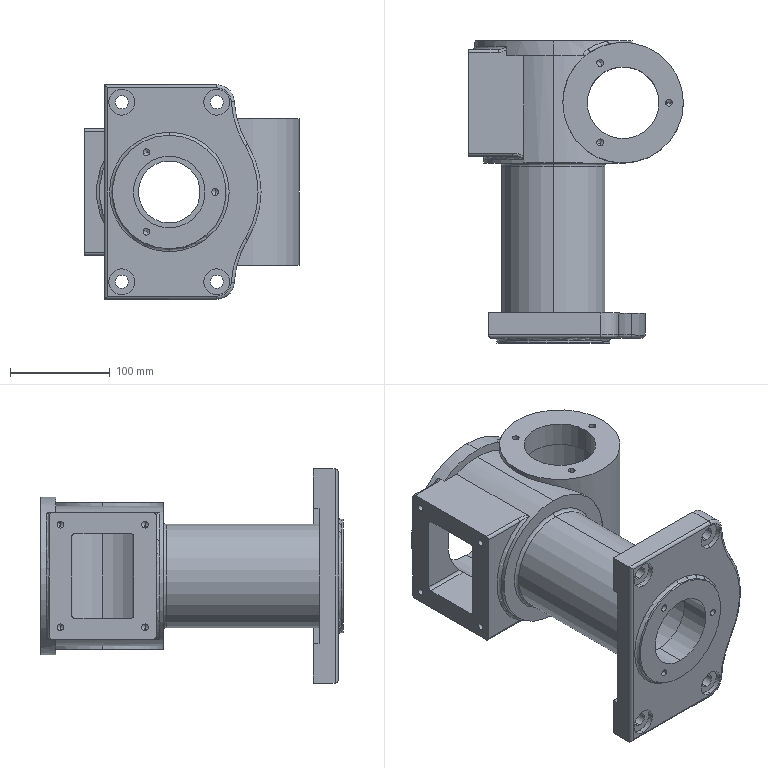Component | SolidWorks | 14-1 | 1 solid | 193 faces | volume 2450873 mm3 | cylinder 100 | cone 38 | plane 35 | torus 11 | spline 9 | commonest cylinder face diameters 6.8 x38 6 x11 13 x8 26 x8 72 x6 104 x4 121 x4 158 x3